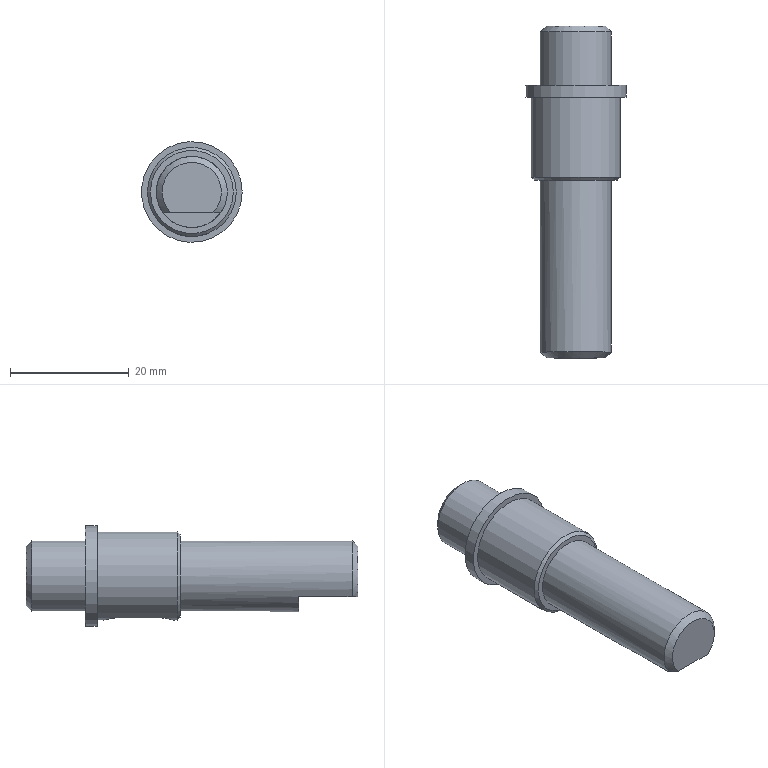Component | NX | CLHKJG_03_OUTPUT_SHAFT | 1 solid | 19 faces | volume 7088 mm3 | plane 10 | cylinder 6 | cone 3 | commonest cylinder face diameters 12 x2 5 x2 17 x1 15 x1